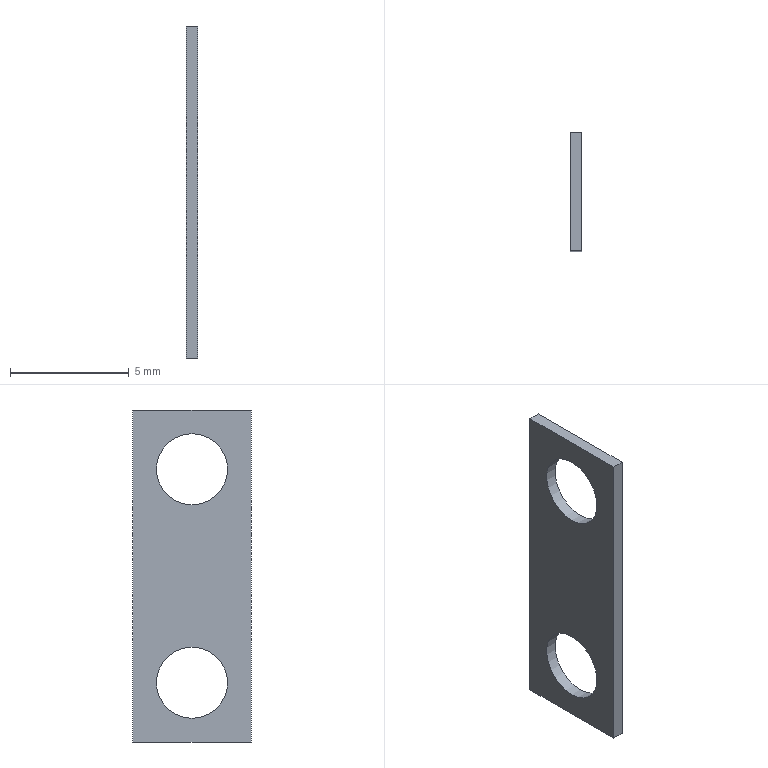Component | NX | AIR_PUMP_PART_01_18 | 1 solid | 8 faces | box 0.5 x 5 x 14 mm | volume 28 mm3 | plane 6 | cylinder 2 | commonest cylinder face diameters 3 x2
STEP:
#1=CARTESIAN_POINT('',(0.,0.,0.));
#2=DIRECTION('',(0.,0.,1.));
#3=DIRECTION('',(1.,0.,0.));
#4=AXIS2_PLACEMENT_3D('',#1,#2,#3);
#5=CARTESIAN_POINT('',(10.001,34.8,36.3));
#6=VERTEX_POINT('',#5);
#7=CARTESIAN_POINT('',(10.001,39.8,36.3));
#8=VERTEX_POINT('',#7);
#9=CARTESIAN_POINT('',(10.001,34.8,36.3));
#10=DIRECTION('',(0.,1.,0.));
#11=VECTOR('',#10,1.);
#12=LINE('',#9,#11);
#13=CARTESIAN_POINT('',(10.501,34.8,36.3));
#14=DIRECTION('',(0.,0.,1.));
#15=DIRECTION('',(1.,0.,0.));
#16=AXIS2_PLACEMENT_3D('',#13,#14,#15);
#17=PLANE('',#16);
#18=CARTESIAN_POINT('',(-0.5,0.));
#19=DIRECTION('',(0.,1.));
#20=VECTOR('',#19,1.);
#21=LINE('',#18,#20);
#22=(GEOMETRIC_REPRESENTATION_CONTEXT(2)PARAMETRIC_REPRESENTATION_CONTEXT()REPRESENTATION_CONTEXT('',''));
#23=DEFINITIONAL_REPRESENTATION('',(#21),#22);
#24=PCURVE('',#17,#23);
#25=CARTESIAN_POINT('',(10.001,37.3,38.8));
#26=DIRECTION('',(-1.,0.,0.));
#27=DIRECTION('',(0.,0.,1.));
#28=AXIS2_PLACEMENT_3D('',#25,#26,#27);
#29=PLANE('',#28);
#30=CARTESIAN_POINT('',(-2.5,-2.5));
#31=DIRECTION('',(0.,1.));
#32=VECTOR('',#31,1.);
#33=LINE('',#30,#32);
#34=(GEOMETRIC_REPRESENTATION_CONTEXT(2)PARAMETRIC_REPRESENTATION_CONTEXT()REPRESENTATION_CONTEXT('',''));
#35=DEFINITIONAL_REPRESENTATION('',(#33),#34);
#36=PCURVE('',#29,#35);
#37=SURFACE_CURVE('',#12,(#24,#36),.PCURVE_S1.);
#38=EDGE_CURVE('',#6,#8,#37,.T.);
#39=ORIENTED_EDGE('',*,*,#38,.T.);
#40=CARTESIAN_POINT('',(10.501,39.8,36.3));
#41=VERTEX_POINT('',#40);
#42=CARTESIAN_POINT('',(10.501,39.8,36.3));
#43=DIRECTION('',(-1.,0.,0.));
#44=VECTOR('',#43,1.);
#45=LINE('',#42,#44);
#46=CARTESIAN_POINT('',(0.,5.));
#47=DIRECTION('',(-1.,0.));
#48=VECTOR('',#47,1.);
#49=LINE('',#46,#48);
#50=(GEOMETRIC_REPRESENTATION_CONTEXT(2)PARAMETRIC_REPRESENTATION_CONTEXT()REPRESENTATION_CONTEXT('',''));
#51=DEFINITIONAL_REPRESENTATION('',(#49),#50);
#52=PCURVE('',#17,#51);
#53=CARTESIAN_POINT('',(10.501,39.8,36.3));
#54=DIRECTION('',(0.,-1.,0.));
#55=DIRECTION('',(-1.,0.,0.));
#56=AXIS2_PLACEMENT_3D('',#53,#54,#55);
#57=PLANE('',#56);
#58=CARTESIAN_POINT('',(0.,0.));
#59=DIRECTION('',(1.,0.));
#60=VECTOR('',#59,1.);
#61=LINE('',#58,#60);
#62=(GEOMETRIC_REPRESENTATION_CONTEXT(2)PARAMETRIC_REPRESENTATION_CONTEXT()REPRESENTATION_CONTEXT('',''));
#63=DEFINITIONAL_REPRESENTATION('',(#61),#62);
#64=PCURVE('',#57,#63);
#65=SURFACE_CURVE('',#45,(#52,#64),.PCURVE_S1.);
#66=EDGE_CURVE('',#41,#8,#65,.T.);
#67=ORIENTED_EDGE('',*,*,#66,.F.);
#68=CARTESIAN_POINT('',(10.501,34.8,36.3));
#69=VERTEX_POINT('',#68);
#70=CARTESIAN_POINT('',(10.501,34.8,36.3));
#71=DIRECTION('',(0.,1.,0.));
#72=VECTOR('',#71,1.);
#73=LINE('',#70,#72);
#74=CARTESIAN_POINT('',(0.,0.));
#75=DIRECTION('',(0.,1.));
#76=VECTOR('',#75,1.);
#77=LINE('',#74,#76);
#78=(GEOMETRIC_REPRESENTATION_CONTEXT(2)PARAMETRIC_REPRESENTATION_CONTEXT()REPRESENTATION_CONTEXT('',''));
#79=DEFINITIONAL_REPRESENTATION('',(#77),#78);
#80=PCURVE('',#17,#79);
#81=CARTESIAN_POINT('',(10.501,37.3,38.8));
#82=DIRECTION('',(-1.,0.,0.));
#83=DIRECTION('',(0.,0.,1.));
#84=AXIS2_PLACEMENT_3D('',#81,#82,#83);
#85=PLANE('',#84);
#86=CARTESIAN_POINT('',(-2.5,-2.5));
#87=DIRECTION('',(0.,1.));
#88=VECTOR('',#87,1.);
#89=LINE('',#86,#88);
#90=(GEOMETRIC_REPRESENTATION_CONTEXT(2)PARAMETRIC_REPRESENTATION_CONTEXT()REPRESENTATION_CONTEXT('',''));
#91=DEFINITIONAL_REPRESENTATION('',(#89),#90);
#92=PCURVE('',#85,#91);
#93=SURFACE_CURVE('',#73,(#80,#92),.PCURVE_S1.);
#94=EDGE_CURVE('',#69,#41,#93,.T.);
#95=ORIENTED_EDGE('',*,*,#94,.F.);
#96=CARTESIAN_POINT('',(10.501,34.8,36.3));
#97=DIRECTION('',(-1.,0.,0.));
#98=VECTOR('',#97,1.);
#99=LINE('',#96,#98);
#100=CARTESIAN_POINT('',(0.,0.));
#101=DIRECTION('',(-1.,0.));
#102=VECTOR('',#101,1.);
#103=LINE('',#100,#102);
#104=(GEOMETRIC_REPRESENTATION_CONTEXT(2)PARAMETRIC_REPRESENTATION_CONTEXT()REPRESENTATION_CONTEXT('',''));
#105=DEFINITIONAL_REPRESENTATION('',(#103),#104);
#106=PCURVE('',#17,#105);
#107=CARTESIAN_POINT('',(10.501,34.8,50.3));
#108=DIRECTION('',(0.,1.,0.));
#109=DIRECTION('',(1.,0.,0.));
#110=AXIS2_PLACEMENT_3D('',#107,#108,#109);
#111=PLANE('',#110);
#112=CARTESIAN_POINT('',(0.,14.));
#113=DIRECTION('',(-1.,0.));
#114=VECTOR('',#113,1.);
#115=LINE('',#112,#114);
#116=(GEOMETRIC_REPRESENTATION_CONTEXT(2)PARAMETRIC_REPRESENTATION_CONTEXT()REPRESENTATION_CONTEXT('',''));
#117=DEFINITIONAL_REPRESENTATION('',(#115),#116);
#118=PCURVE('',#111,#117);
#119=SURFACE_CURVE('',#99,(#106,#118),.PCURVE_S1.);
#120=EDGE_CURVE('',#69,#6,#119,.T.);
#121=ORIENTED_EDGE('',*,*,#120,.T.);
#122=EDGE_LOOP('',(#39,#67,#95,#121));
#123=FACE_BOUND('',#122,.T.);
#124=ADVANCED_FACE('',(#123),#17,.F.);
#125=CARTESIAN_POINT('',(10.001,39.8,50.3));
#126=VERTEX_POINT('',#125);
#127=CARTESIAN_POINT('',(10.001,39.8,36.3));
#128=DIRECTION('',(0.,0.,1.));
#129=VECTOR('',#128,1.);
#130=LINE('',#127,#129);
#131=CARTESIAN_POINT('',(0.5,0.));
#132=DIRECTION('',(0.,-1.));
#133=VECTOR('',#132,1.);
#134=LINE('',#131,#133);
#135=(GEOMETRIC_REPRESENTATION_CONTEXT(2)PARAMETRIC_REPRESENTATION_CONTEXT()REPRESENTATION_CONTEXT('',''));
#136=DEFINITIONAL_REPRESENTATION('',(#134),#135);
#137=PCURVE('',#57,#136);
#138=CARTESIAN_POINT('',(-2.5,2.5));
#139=DIRECTION('',(1.,0.));
#140=VECTOR('',#139,1.);
#141=LINE('',#138,#140);
#142=(GEOMETRIC_REPRESENTATION_CONTEXT(2)PARAMETRIC_REPRESENTATION_CONTEXT()REPRESENTATION_CONTEXT('',''));
#143=DEFINITIONAL_REPRESENTATION('',(#141),#142);
#144=PCURVE('',#29,#143);
#145=SURFACE_CURVE('',#130,(#137,#144),.PCURVE_S1.);
#146=EDGE_CURVE('',#8,#126,#145,.T.);
#147=ORIENTED_EDGE('',*,*,#146,.T.);
#148=CARTESIAN_POINT('',(10.501,39.8,50.3));
#149=VERTEX_POINT('',#148);
#150=CARTESIAN_POINT('',(10.501,39.8,50.3));
#151=DIRECTION('',(-1.,0.,0.));
#152=VECTOR('',#151,1.);
#153=LINE('',#150,#152);
#154=CARTESIAN_POINT('',(0.,-14.));
#155=DIRECTION('',(1.,0.));
#156=VECTOR('',#155,1.);
#157=LINE('',#154,#156);
#158=(GEOMETRIC_REPRESENTATION_CONTEXT(2)PARAMETRIC_REPRESENTATION_CONTEXT()REPRESENTATION_CONTEXT('',''));
#159=DEFINITIONAL_REPRESENTATION('',(#157),#158);
#160=PCURVE('',#57,#159);
#161=CARTESIAN_POINT('',(10.501,39.8,50.3));
#162=DIRECTION('',(0.,0.,-1.));
#163=DIRECTION('',(-1.,0.,0.));
#164=AXIS2_PLACEMENT_3D('',#161,#162,#163);
#165=PLANE('',#164);
#166=CARTESIAN_POINT('',(0.,0.));
#167=DIRECTION('',(1.,0.));
#168=VECTOR('',#167,1.);
#169=LINE('',#166,#168);
#170=(GEOMETRIC_REPRESENTATION_CONTEXT(2)PARAMETRIC_REPRESENTATION_CONTEXT()REPRESENTATION_CONTEXT('',''));
#171=DEFINITIONAL_REPRESENTATION('',(#169),#170);
#172=PCURVE('',#165,#171);
#173=SURFACE_CURVE('',#153,(#160,#172),.PCURVE_S1.);
#174=EDGE_CURVE('',#149,#126,#173,.T.);
#175=ORIENTED_EDGE('',*,*,#174,.F.);
#176=CARTESIAN_POINT('',(10.501,39.8,36.3));
#177=DIRECTION('',(0.,0.,1.));
#178=VECTOR('',#177,1.);
#179=LINE('',#176,#178);
#180=CARTESIAN_POINT('',(0.,0.));
#181=DIRECTION('',(0.,-1.));
#182=VECTOR('',#181,1.);
#183=LINE('',#180,#182);
#184=(GEOMETRIC_REPRESENTATION_CONTEXT(2)PARAMETRIC_REPRESENTATION_CONTEXT()REPRESENTATION_CONTEXT('',''));
#185=DEFINITIONAL_REPRESENTATION('',(#183),#184);
#186=PCURVE('',#57,#185);
#187=CARTESIAN_POINT('',(-2.5,2.5));
#188=DIRECTION('',(1.,0.));
#189=VECTOR('',#188,1.);
#190=LINE('',#187,#189);
#191=(GEOMETRIC_REPRESENTATION_CONTEXT(2)PARAMETRIC_REPRESENTATION_CONTEXT()REPRESENTATION_CONTEXT('',''));
#192=DEFINITIONAL_REPRESENTATION('',(#190),#191);
#193=PCURVE('',#85,#192);
#194=SURFACE_CURVE('',#179,(#186,#193),.PCURVE_S1.);
#195=EDGE_CURVE('',#41,#149,#194,.T.);
#196=ORIENTED_EDGE('',*,*,#195,.F.);
#197=ORIENTED_EDGE('',*,*,#66,.T.);
#198=EDGE_LOOP('',(#147,#175,#196,#197));
#199=FACE_BOUND('',#198,.T.);
#200=ADVANCED_FACE('',(#199),#57,.F.);
#201=CARTESIAN_POINT('',(10.001,34.8,50.3));
#202=VERTEX_POINT('',#201);
#203=CARTESIAN_POINT('',(10.001,39.8,50.3));
#204=DIRECTION('',(0.,-1.,0.));
#205=VECTOR('',#204,1.);
#206=LINE('',#203,#205);
#207=CARTESIAN_POINT('',(0.5,0.));
#208=DIRECTION('',(0.,-1.));
#209=VECTOR('',#208,1.);
#210=LINE('',#207,#209);
#211=(GEOMETRIC_REPRESENTATION_CONTEXT(2)PARAMETRIC_REPRESENTATION_CONTEXT()REPRESENTATION_CONTEXT('',''));
#212=DEFINITIONAL_REPRESENTATION('',(#210),#211);
#213=PCURVE('',#165,#212);
#214=CARTESIAN_POINT('',(11.5,2.5));
#215=DIRECTION('',(0.,-1.));
#216=VECTOR('',#215,1.);
#217=LINE('',#214,#216);
#218=(GEOMETRIC_REPRESENTATION_CONTEXT(2)PARAMETRIC_REPRESENTATION_CONTEXT()REPRESENTATION_CONTEXT('',''));
#219=DEFINITIONAL_REPRESENTATION('',(#217),#218);
#220=PCURVE('',#29,#219);
#221=SURFACE_CURVE('',#206,(#213,#220),.PCURVE_S1.);
#222=EDGE_CURVE('',#126,#202,#221,.T.);
#223=ORIENTED_EDGE('',*,*,#222,.T.);
#224=CARTESIAN_POINT('',(10.501,34.8,50.3));
#225=VERTEX_POINT('',#224);
#226=CARTESIAN_POINT('',(10.501,34.8,50.3));
#227=DIRECTION('',(-1.,0.,0.));
#228=VECTOR('',#227,1.);
#229=LINE('',#226,#228);
#230=CARTESIAN_POINT('',(0.,-5.));
#231=DIRECTION('',(1.,0.));
#232=VECTOR('',#231,1.);
#233=LINE('',#230,#232);
#234=(GEOMETRIC_REPRESENTATION_CONTEXT(2)PARAMETRIC_REPRESENTATION_CONTEXT()REPRESENTATION_CONTEXT('',''));
#235=DEFINITIONAL_REPRESENTATION('',(#233),#234);
#236=PCURVE('',#165,#235);
#237=CARTESIAN_POINT('',(0.,0.));
#238=DIRECTION('',(-1.,0.));
#239=VECTOR('',#238,1.);
#240=LINE('',#237,#239);
#241=(GEOMETRIC_REPRESENTATION_CONTEXT(2)PARAMETRIC_REPRESENTATION_CONTEXT()REPRESENTATION_CONTEXT('',''));
#242=DEFINITIONAL_REPRESENTATION('',(#240),#241);
#243=PCURVE('',#111,#242);
#244=SURFACE_CURVE('',#229,(#236,#243),.PCURVE_S1.);
#245=EDGE_CURVE('',#225,#202,#244,.T.);
#246=ORIENTED_EDGE('',*,*,#245,.F.);
#247=CARTESIAN_POINT('',(10.501,39.8,50.3));
#248=DIRECTION('',(0.,-1.,0.));
#249=VECTOR('',#248,1.);
#250=LINE('',#247,#249);
#251=CARTESIAN_POINT('',(0.,0.));
#252=DIRECTION('',(0.,-1.));
#253=VECTOR('',#252,1.);
#254=LINE('',#251,#253);
#255=(GEOMETRIC_REPRESENTATION_CONTEXT(2)PARAMETRIC_REPRESENTATION_CONTEXT()REPRESENTATION_CONTEXT('',''));
#256=DEFINITIONAL_REPRESENTATION('',(#254),#255);
#257=PCURVE('',#165,#256);
#258=CARTESIAN_POINT('',(11.5,2.5));
#259=DIRECTION('',(0.,-1.));
#260=VECTOR('',#259,1.);
#261=LINE('',#258,#260);
#262=(GEOMETRIC_REPRESENTATION_CONTEXT(2)PARAMETRIC_REPRESENTATION_CONTEXT()REPRESENTATION_CONTEXT('',''));
#263=DEFINITIONAL_REPRESENTATION('',(#261),#262);
#264=PCURVE('',#85,#263);
#265=SURFACE_CURVE('',#250,(#257,#264),.PCURVE_S1.);
#266=EDGE_CURVE('',#149,#225,#265,.T.);
#267=ORIENTED_EDGE('',*,*,#266,.F.);
#268=ORIENTED_EDGE('',*,*,#174,.T.);
#269=EDGE_LOOP('',(#223,#246,#267,#268));
#270=FACE_BOUND('',#269,.T.);
#271=ADVANCED_FACE('',(#270),#165,.F.);
#272=CARTESIAN_POINT('',(10.501,37.3,40.3));
#273=VERTEX_POINT('',#272);
#274=CARTESIAN_POINT('',(10.501,37.3,38.8));
#275=DIRECTION('',(-1.,0.,0.));
#276=DIRECTION('',(0.,0.,1.));
#277=AXIS2_PLACEMENT_3D('',#274,#275,#276);
#278=CIRCLE('',#277,1.5);
#279=CARTESIAN_POINT('',(10.501,37.3,38.8));
#280=DIRECTION('',(-1.,0.,0.));
#281=DIRECTION('',(0.,0.,1.));
#282=AXIS2_PLACEMENT_3D('',#279,#280,#281);
#283=CYLINDRICAL_SURFACE('',#282,1.5);
#284=CARTESIAN_POINT('',(0.,0.));
#285=DIRECTION('',(1.,0.));
#286=VECTOR('',#285,1.);
#287=LINE('',#284,#286);
#288=(GEOMETRIC_REPRESENTATION_CONTEXT(2)PARAMETRIC_REPRESENTATION_CONTEXT()REPRESENTATION_CONTEXT('',''));
#289=DEFINITIONAL_REPRESENTATION('',(#287),#288);
#290=PCURVE('',#283,#289);
#291=CARTESIAN_POINT('',(0.,0.));
#292=DIRECTION('',(1.,0.));
#293=AXIS2_PLACEMENT_2D('',#291,#292);
#294=CIRCLE('',#293,1.5);
#295=(GEOMETRIC_REPRESENTATION_CONTEXT(2)PARAMETRIC_REPRESENTATION_CONTEXT()REPRESENTATION_CONTEXT('',''));
#296=DEFINITIONAL_REPRESENTATION('',(#294),#295);
#297=PCURVE('',#85,#296);
#298=SURFACE_CURVE('',#278,(#290,#297),.PCURVE_S1.);
#299=EDGE_CURVE('',#273,#273,#298,.T.);
#300=ORIENTED_EDGE('',*,*,#299,.T.);
#301=CARTESIAN_POINT('',(10.001,37.3,40.3));
#302=VERTEX_POINT('',#301);
#303=CARTESIAN_POINT('',(10.501,37.3,40.3));
#304=CARTESIAN_POINT('',(10.001,37.3,40.3));
#305=B_SPLINE_CURVE_WITH_KNOTS('',1,(#303,#304),.UNSPECIFIED.,.F.,.F.,(2,2),(0.,0.5),.PIECEWISE_BEZIER_KNOTS.);
#306=CARTESIAN_POINT('',(6.283,0.));
#307=DIRECTION('',(0.,1.));
#308=VECTOR('',#307,1.);
#309=LINE('',#306,#308);
#310=(GEOMETRIC_REPRESENTATION_CONTEXT(2)PARAMETRIC_REPRESENTATION_CONTEXT()REPRESENTATION_CONTEXT('',''));
#311=DEFINITIONAL_REPRESENTATION('',(#309),#310);
#312=PCURVE('',#283,#311);
#313=CARTESIAN_POINT('',(0.,0.));
#314=DIRECTION('',(0.,1.));
#315=VECTOR('',#314,1.);
#316=LINE('',#313,#315);
#317=(GEOMETRIC_REPRESENTATION_CONTEXT(2)PARAMETRIC_REPRESENTATION_CONTEXT()REPRESENTATION_CONTEXT('',''));
#318=DEFINITIONAL_REPRESENTATION('',(#316),#317);
#319=PCURVE('',#283,#318);
#320=SEAM_CURVE('',#305,(#312,#319),.PCURVE_S1.);
#321=EDGE_CURVE('',#273,#302,#320,.T.);
#322=ORIENTED_EDGE('',*,*,#321,.T.);
#323=CARTESIAN_POINT('',(10.001,37.3,38.8));
#324=DIRECTION('',(-1.,0.,0.));
#325=DIRECTION('',(0.,0.,1.));
#326=AXIS2_PLACEMENT_3D('',#323,#324,#325);
#327=CIRCLE('',#326,1.5);
#328=CARTESIAN_POINT('',(0.,0.5));
#329=DIRECTION('',(1.,0.));
#330=VECTOR('',#329,1.);
#331=LINE('',#328,#330);
#332=(GEOMETRIC_REPRESENTATION_CONTEXT(2)PARAMETRIC_REPRESENTATION_CONTEXT()REPRESENTATION_CONTEXT('',''));
#333=DEFINITIONAL_REPRESENTATION('',(#331),#332);
#334=PCURVE('',#283,#333);
#335=CARTESIAN_POINT('',(0.,0.));
#336=DIRECTION('',(1.,0.));
#337=AXIS2_PLACEMENT_2D('',#335,#336);
#338=CIRCLE('',#337,1.5);
#339=(GEOMETRIC_REPRESENTATION_CONTEXT(2)PARAMETRIC_REPRESENTATION_CONTEXT()REPRESENTATION_CONTEXT('',''));
#340=DEFINITIONAL_REPRESENTATION('',(#338),#339);
#341=PCURVE('',#29,#340);
#342=SURFACE_CURVE('',#327,(#334,#341),.PCURVE_S1.);
#343=EDGE_CURVE('',#302,#302,#342,.T.);
#344=ORIENTED_EDGE('',*,*,#343,.F.);
#345=ORIENTED_EDGE('',*,*,#321,.F.);
#346=EDGE_LOOP('',(#300,#322,#344,#345));
#347=FACE_BOUND('',#346,.F.);
#348=ADVANCED_FACE('',(#347),#283,.F.);
#349=CARTESIAN_POINT('',(10.001,34.8,50.3));
#350=DIRECTION('',(0.,0.,-1.));
#351=VECTOR('',#350,1.);
#352=LINE('',#349,#351);
#353=CARTESIAN_POINT('',(-0.5,0.));
#354=DIRECTION('',(0.,1.));
#355=VECTOR('',#354,1.);
#356=LINE('',#353,#355);
#357=(GEOMETRIC_REPRESENTATION_CONTEXT(2)PARAMETRIC_REPRESENTATION_CONTEXT()REPRESENTATION_CONTEXT('',''));
#358=DEFINITIONAL_REPRESENTATION('',(#356),#357);
#359=PCURVE('',#111,#358);
#360=CARTESIAN_POINT('',(11.5,-2.5));
#361=DIRECTION('',(-1.,0.));
#362=VECTOR('',#361,1.);
#363=LINE('',#360,#362);
#364=(GEOMETRIC_REPRESENTATION_CONTEXT(2)PARAMETRIC_REPRESENTATION_CONTEXT()REPRESENTATION_CONTEXT('',''));
#365=DEFINITIONAL_REPRESENTATION('',(#363),#364);
#366=PCURVE('',#29,#365);
#367=SURFACE_CURVE('',#352,(#359,#366),.PCURVE_S1.);
#368=EDGE_CURVE('',#202,#6,#367,.T.);
#369=ORIENTED_EDGE('',*,*,#368,.T.);
#370=ORIENTED_EDGE('',*,*,#120,.F.);
#371=CARTESIAN_POINT('',(10.501,34.8,50.3));
#372=DIRECTION('',(0.,0.,-1.));
#373=VECTOR('',#372,1.);
#374=LINE('',#371,#373);
#375=CARTESIAN_POINT('',(0.,0.));
#376=DIRECTION('',(0.,1.));
#377=VECTOR('',#376,1.);
#378=LINE('',#375,#377);
#379=(GEOMETRIC_REPRESENTATION_CONTEXT(2)PARAMETRIC_REPRESENTATION_CONTEXT()REPRESENTATION_CONTEXT('',''));
#380=DEFINITIONAL_REPRESENTATION('',(#378),#379);
#381=PCURVE('',#111,#380);
#382=CARTESIAN_POINT('',(11.5,-2.5));
#383=DIRECTION('',(-1.,0.));
#384=VECTOR('',#383,1.);
#385=LINE('',#382,#384);
#386=(GEOMETRIC_REPRESENTATION_CONTEXT(2)PARAMETRIC_REPRESENTATION_CONTEXT()REPRESENTATION_CONTEXT('',''));
#387=DEFINITIONAL_REPRESENTATION('',(#385),#386);
#388=PCURVE('',#85,#387);
#389=SURFACE_CURVE('',#374,(#381,#388),.PCURVE_S1.);
#390=EDGE_CURVE('',#225,#69,#389,.T.);
#391=ORIENTED_EDGE('',*,*,#390,.F.);
#392=ORIENTED_EDGE('',*,*,#245,.T.);
#393=EDGE_LOOP('',(#369,#370,#391,#392));
#394=FACE_BOUND('',#393,.T.);
#395=ADVANCED_FACE('',(#394),#111,.F.);
#396=CARTESIAN_POINT('',(10.501,37.3,46.3));
#397=VERTEX_POINT('',#396);
#398=CARTESIAN_POINT('',(10.501,37.3,47.8));
#399=DIRECTION('',(1.,0.,0.));
#400=DIRECTION('',(0.,0.,-1.));
#401=AXIS2_PLACEMENT_3D('',#398,#399,#400);
#402=CIRCLE('',#401,1.5);
#403=CARTESIAN_POINT('',(10.501,37.3,47.8));
#404=DIRECTION('',(-1.,0.,0.));
#405=DIRECTION('',(0.,0.,1.));
#406=AXIS2_PLACEMENT_3D('',#403,#404,#405);
#407=CYLINDRICAL_SURFACE('',#406,1.5);
#408=CARTESIAN_POINT('',(9.425,0.));
#409=DIRECTION('',(-1.,0.));
#410=VECTOR('',#409,1.);
#411=LINE('',#408,#410);
#412=(GEOMETRIC_REPRESENTATION_CONTEXT(2)PARAMETRIC_REPRESENTATION_CONTEXT()REPRESENTATION_CONTEXT('',''));
#413=DEFINITIONAL_REPRESENTATION('',(#411),#412);
#414=PCURVE('',#407,#413);
#415=CARTESIAN_POINT('',(7.5,0.));
#416=CARTESIAN_POINT('',(7.5,2.598));
#417=CARTESIAN_POINT('',(9.75,1.299));
#418=CARTESIAN_POINT('',(12.,0.));
#419=CARTESIAN_POINT('',(9.75,-1.299));
#420=CARTESIAN_POINT('',(7.5,-2.598));
#421=CARTESIAN_POINT('',(7.5,0.));
#422=(BOUNDED_CURVE()B_SPLINE_CURVE(2,(#415,#416,#417,#418,#419,#420,#421),.UNSPECIFIED.,.T.,.F.)B_SPLINE_CURVE_WITH_KNOTS((1,2,2,2,2,1),(-2.094,0.,2.094,4.189,6.283,8.378),.UNSPECIFIED.)CURVE()GEOMETRIC_REPRESENTATION_ITEM()RATIONAL_B_SPLINE_CURVE((1.,0.5,1.,0.5,1.,0.5,1.))REPRESENTATION_ITEM(''));
#423=(GEOMETRIC_REPRESENTATION_CONTEXT(2)PARAMETRIC_REPRESENTATION_CONTEXT()REPRESENTATION_CONTEXT('',''));
#424=DEFINITIONAL_REPRESENTATION('',(#422),#423);
#425=PCURVE('',#85,#424);
#426=SURFACE_CURVE('',#402,(#414,#425),.PCURVE_S1.);
#427=EDGE_CURVE('',#397,#397,#426,.T.);
#428=ORIENTED_EDGE('',*,*,#427,.F.);
#429=CARTESIAN_POINT('',(10.001,37.3,46.3));
#430=VERTEX_POINT('',#429);
#431=CARTESIAN_POINT('',(10.501,37.3,46.3));
#432=CARTESIAN_POINT('',(10.001,37.3,46.3));
#433=B_SPLINE_CURVE_WITH_KNOTS('',1,(#431,#432),.UNSPECIFIED.,.F.,.F.,(2,2),(0.,0.5),.PIECEWISE_BEZIER_KNOTS.);
#434=CARTESIAN_POINT('',(9.425,0.));
#435=DIRECTION('',(0.,1.));
#436=VECTOR('',#435,1.);
#437=LINE('',#434,#436);
#438=(GEOMETRIC_REPRESENTATION_CONTEXT(2)PARAMETRIC_REPRESENTATION_CONTEXT()REPRESENTATION_CONTEXT('',''));
#439=DEFINITIONAL_REPRESENTATION('',(#437),#438);
#440=PCURVE('',#407,#439);
#441=CARTESIAN_POINT('',(3.142,0.));
#442=DIRECTION('',(0.,1.));
#443=VECTOR('',#442,1.);
#444=LINE('',#441,#443);
#445=(GEOMETRIC_REPRESENTATION_CONTEXT(2)PARAMETRIC_REPRESENTATION_CONTEXT()REPRESENTATION_CONTEXT('',''));
#446=DEFINITIONAL_REPRESENTATION('',(#444),#445);
#447=PCURVE('',#407,#446);
#448=SEAM_CURVE('',#433,(#440,#447),.PCURVE_S1.);
#449=EDGE_CURVE('',#397,#430,#448,.T.);
#450=ORIENTED_EDGE('',*,*,#449,.T.);
#451=CARTESIAN_POINT('',(10.001,37.3,47.8));
#452=DIRECTION('',(1.,0.,0.));
#453=DIRECTION('',(0.,0.,-1.));
#454=AXIS2_PLACEMENT_3D('',#451,#452,#453);
#455=CIRCLE('',#454,1.5);
#456=CARTESIAN_POINT('',(9.425,0.5));
#457=DIRECTION('',(-1.,0.));
#458=VECTOR('',#457,1.);
#459=LINE('',#456,#458);
#460=(GEOMETRIC_REPRESENTATION_CONTEXT(2)PARAMETRIC_REPRESENTATION_CONTEXT()REPRESENTATION_CONTEXT('',''));
#461=DEFINITIONAL_REPRESENTATION('',(#459),#460);
#462=PCURVE('',#407,#461);
#463=CARTESIAN_POINT('',(7.5,0.));
#464=CARTESIAN_POINT('',(7.5,2.598));
#465=CARTESIAN_POINT('',(9.75,1.299));
#466=CARTESIAN_POINT('',(12.,0.));
#467=CARTESIAN_POINT('',(9.75,-1.299));
#468=CARTESIAN_POINT('',(7.5,-2.598));
#469=CARTESIAN_POINT('',(7.5,0.));
#470=(BOUNDED_CURVE()B_SPLINE_CURVE(2,(#463,#464,#465,#466,#467,#468,#469),.UNSPECIFIED.,.T.,.F.)B_SPLINE_CURVE_WITH_KNOTS((1,2,2,2,2,1),(-2.094,0.,2.094,4.189,6.283,8.378),.UNSPECIFIED.)CURVE()GEOMETRIC_REPRESENTATION_ITEM()RATIONAL_B_SPLINE_CURVE((1.,0.5,1.,0.5,1.,0.5,1.))REPRESENTATION_ITEM(''));
#471=(GEOMETRIC_REPRESENTATION_CONTEXT(2)PARAMETRIC_REPRESENTATION_CONTEXT()REPRESENTATION_CONTEXT('',''));
#472=DEFINITIONAL_REPRESENTATION('',(#470),#471);
#473=PCURVE('',#29,#472);
#474=SURFACE_CURVE('',#455,(#462,#473),.PCURVE_S1.);
#475=EDGE_CURVE('',#430,#430,#474,.T.);
#476=ORIENTED_EDGE('',*,*,#475,.T.);
#477=ORIENTED_EDGE('',*,*,#449,.F.);
#478=EDGE_LOOP('',(#428,#450,#476,#477));
#479=FACE_BOUND('',#478,.F.);
#480=ADVANCED_FACE('',(#479),#407,.F.);
#481=ORIENTED_EDGE('',*,*,#94,.T.);
#482=ORIENTED_EDGE('',*,*,#195,.T.);
#483=ORIENTED_EDGE('',*,*,#266,.T.);
#484=ORIENTED_EDGE('',*,*,#390,.T.);
#485=EDGE_LOOP('',(#481,#482,#483,#484));
#486=FACE_BOUND('',#485,.T.);
#487=ORIENTED_EDGE('',*,*,#299,.T.);
#488=EDGE_LOOP('',(#487));
#489=FACE_BOUND('',#488,.T.);
#490=ORIENTED_EDGE('',*,*,#427,.F.);
#491=EDGE_LOOP('',(#490));
#492=FACE_BOUND('',#491,.T.);
#493=ADVANCED_FACE('',(#486,#489,#492),#85,.F.);
#494=ORIENTED_EDGE('',*,*,#38,.F.);
#495=ORIENTED_EDGE('',*,*,#368,.F.);
#496=ORIENTED_EDGE('',*,*,#222,.F.);
#497=ORIENTED_EDGE('',*,*,#146,.F.);
#498=EDGE_LOOP('',(#494,#495,#496,#497));
#499=FACE_BOUND('',#498,.T.);
#500=ORIENTED_EDGE('',*,*,#343,.F.);
#501=EDGE_LOOP('',(#500));
#502=FACE_BOUND('',#501,.T.);
#503=ORIENTED_EDGE('',*,*,#475,.T.);
#504=EDGE_LOOP('',(#503));
#505=FACE_BOUND('',#504,.T.);
#506=ADVANCED_FACE('',(#499,#502,#505),#29,.T.);
#507=CLOSED_SHELL('',(#124,#200,#271,#348,#395,#480,#493,#506));
#508=MANIFOLD_SOLID_BREP('',#507);
#509=(LENGTH_UNIT()NAMED_UNIT(*)SI_UNIT(.MILLI.,.METRE.));
#510=UNCERTAINTY_MEASURE_WITH_UNIT(LENGTH_MEASURE(0.000002),#509,'','');
#511=(NAMED_UNIT(*)PLANE_ANGLE_UNIT()SI_UNIT($,.RADIAN.));
#512=(NAMED_UNIT(*)SI_UNIT($,.STERADIAN.)SOLID_ANGLE_UNIT());
#513=(GEOMETRIC_REPRESENTATION_CONTEXT(3)GLOBAL_UNCERTAINTY_ASSIGNED_CONTEXT((#510))GLOBAL_UNIT_ASSIGNED_CONTEXT((#509,#511,#512))REPRESENTATION_CONTEXT('',''));
#514=ADVANCED_BREP_SHAPE_REPRESENTATION('',(#4,#508),#513);